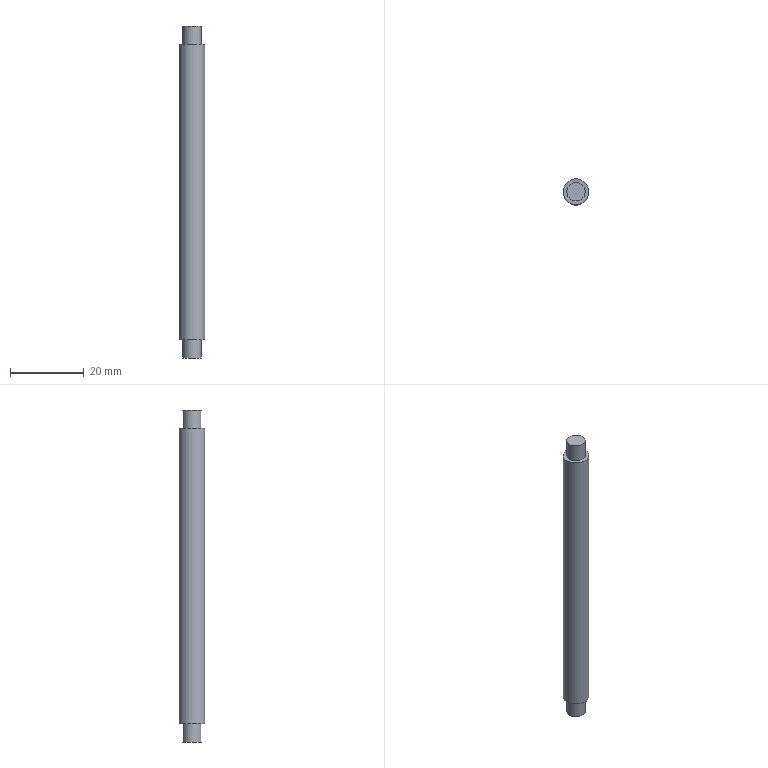Component | NX | STRUT_3 | 1 solid | 7 faces | box 7 x 7 x 90 mm | volume 3275 mm3 | plane 4 | cylinder 3 | commonest cylinder face diameters 5 x2 7 x1
STEP:
#1=CARTESIAN_POINT('',(0.,0.,0.));
#2=DIRECTION('',(0.,0.,1.));
#3=DIRECTION('',(1.,0.,0.));
#4=AXIS2_PLACEMENT_3D('',#1,#2,#3);
#5=CARTESIAN_POINT('',(-7.112,-26.214,-154.808));
#6=VERTEX_POINT('',#5);
#7=CARTESIAN_POINT('',(-9.612,-26.214,-154.808));
#8=DIRECTION('',(0.,0.,1.));
#9=DIRECTION('',(1.,0.,0.));
#10=AXIS2_PLACEMENT_3D('',#7,#8,#9);
#11=CIRCLE('',#10,2.5);
#12=CARTESIAN_POINT('',(-9.612,-26.214,-154.808));
#13=DIRECTION('',(0.,0.,-1.));
#14=DIRECTION('',(-1.,0.,0.));
#15=AXIS2_PLACEMENT_3D('',#12,#13,#14);
#16=PLANE('',#15);
#17=CARTESIAN_POINT('',(-2.5,0.));
#18=CARTESIAN_POINT('',(-2.5,4.33));
#19=CARTESIAN_POINT('',(1.25,2.165));
#20=CARTESIAN_POINT('',(5.,0.));
#21=CARTESIAN_POINT('',(1.25,-2.165));
#22=CARTESIAN_POINT('',(-2.5,-4.33));
#23=CARTESIAN_POINT('',(-2.5,0.));
#24=(BOUNDED_CURVE()B_SPLINE_CURVE(2,(#17,#18,#19,#20,#21,#22,#23),.UNSPECIFIED.,.T.,.F.)B_SPLINE_CURVE_WITH_KNOTS((1,2,2,2,2,1),(-2.094,0.,2.094,4.189,6.283,8.378),.UNSPECIFIED.)CURVE()GEOMETRIC_REPRESENTATION_ITEM()RATIONAL_B_SPLINE_CURVE((1.,0.5,1.,0.5,1.,0.5,1.))REPRESENTATION_ITEM(''));
#25=(GEOMETRIC_REPRESENTATION_CONTEXT(2)PARAMETRIC_REPRESENTATION_CONTEXT()REPRESENTATION_CONTEXT('',''));
#26=DEFINITIONAL_REPRESENTATION('',(#24),#25);
#27=PCURVE('',#16,#26);
#28=CARTESIAN_POINT('',(-9.612,-26.214,-154.808));
#29=DIRECTION('',(0.,0.,1.));
#30=DIRECTION('',(1.,0.,0.));
#31=AXIS2_PLACEMENT_3D('',#28,#29,#30);
#32=CYLINDRICAL_SURFACE('',#31,2.5);
#33=CARTESIAN_POINT('',(0.,0.));
#34=DIRECTION('',(1.,0.));
#35=VECTOR('',#34,1.);
#36=LINE('',#33,#35);
#37=(GEOMETRIC_REPRESENTATION_CONTEXT(2)PARAMETRIC_REPRESENTATION_CONTEXT()REPRESENTATION_CONTEXT('',''));
#38=DEFINITIONAL_REPRESENTATION('',(#36),#37);
#39=PCURVE('',#32,#38);
#40=SURFACE_CURVE('',#11,(#27,#39),.PCURVE_S1.);
#41=EDGE_CURVE('',#6,#6,#40,.T.);
#42=ORIENTED_EDGE('',*,*,#41,.F.);
#43=EDGE_LOOP('',(#42));
#44=FACE_BOUND('',#43,.T.);
#45=ADVANCED_FACE('',(#44),#16,.T.);
#46=CARTESIAN_POINT('',(-7.112,-26.214,-149.808));
#47=VERTEX_POINT('',#46);
#48=CARTESIAN_POINT('',(-12.112,-26.214,-149.808));
#49=VERTEX_POINT('',#48);
#50=CARTESIAN_POINT('',(-9.612,-26.214,-149.808));
#51=DIRECTION('',(0.,0.,1.));
#52=DIRECTION('',(-1.,0.,0.));
#53=AXIS2_PLACEMENT_3D('',#50,#51,#52);
#54=CIRCLE('',#53,2.5);
#55=CARTESIAN_POINT('',(-3.142,5.));
#56=DIRECTION('',(1.,0.));
#57=VECTOR('',#56,1.);
#58=LINE('',#55,#57);
#59=(GEOMETRIC_REPRESENTATION_CONTEXT(2)PARAMETRIC_REPRESENTATION_CONTEXT()REPRESENTATION_CONTEXT('',''));
#60=DEFINITIONAL_REPRESENTATION('',(#58),#59);
#61=PCURVE('',#32,#60);
#62=CARTESIAN_POINT('',(-9.612,-26.214,-149.808));
#63=DIRECTION('',(0.,0.,-1.));
#64=DIRECTION('',(-1.,0.,0.));
#65=AXIS2_PLACEMENT_3D('',#62,#63,#64);
#66=PLANE('',#65);
#67=CARTESIAN_POINT('',(2.5,0.));
#68=CARTESIAN_POINT('',(2.5,-4.33));
#69=CARTESIAN_POINT('',(-1.25,-2.165));
#70=CARTESIAN_POINT('',(-5.,-0.));
#71=CARTESIAN_POINT('',(-1.25,2.165));
#72=CARTESIAN_POINT('',(2.5,4.33));
#73=CARTESIAN_POINT('',(2.5,0.));
#74=(BOUNDED_CURVE()B_SPLINE_CURVE(2,(#67,#68,#69,#70,#71,#72,#73),.UNSPECIFIED.,.T.,.F.)B_SPLINE_CURVE_WITH_KNOTS((1,2,2,2,2,1),(-2.094,0.,2.094,4.189,6.283,8.378),.UNSPECIFIED.)CURVE()GEOMETRIC_REPRESENTATION_ITEM()RATIONAL_B_SPLINE_CURVE((1.,0.5,1.,0.5,1.,0.5,1.))REPRESENTATION_ITEM(''));
#75=(GEOMETRIC_REPRESENTATION_CONTEXT(2)PARAMETRIC_REPRESENTATION_CONTEXT()REPRESENTATION_CONTEXT('',''));
#76=DEFINITIONAL_REPRESENTATION('',(#74),#75);
#77=PCURVE('',#66,#76);
#78=SURFACE_CURVE('',#54,(#61,#77),.PCURVE_S1.);
#79=EDGE_CURVE('',#47,#49,#78,.T.);
#80=ORIENTED_EDGE('',*,*,#79,.F.);
#81=CARTESIAN_POINT('',(-7.112,-26.214,-154.808));
#82=CARTESIAN_POINT('',(-7.112,-26.214,-149.808));
#83=B_SPLINE_CURVE_WITH_KNOTS('',1,(#81,#82),.UNSPECIFIED.,.F.,.F.,(2,2),(0.,5.),.PIECEWISE_BEZIER_KNOTS.);
#84=CARTESIAN_POINT('',(0.,0.));
#85=DIRECTION('',(0.,1.));
#86=VECTOR('',#85,1.);
#87=LINE('',#84,#86);
#88=(GEOMETRIC_REPRESENTATION_CONTEXT(2)PARAMETRIC_REPRESENTATION_CONTEXT()REPRESENTATION_CONTEXT('',''));
#89=DEFINITIONAL_REPRESENTATION('',(#87),#88);
#90=PCURVE('',#32,#89);
#91=CARTESIAN_POINT('',(6.283,0.));
#92=DIRECTION('',(0.,1.));
#93=VECTOR('',#92,1.);
#94=LINE('',#91,#93);
#95=(GEOMETRIC_REPRESENTATION_CONTEXT(2)PARAMETRIC_REPRESENTATION_CONTEXT()REPRESENTATION_CONTEXT('',''));
#96=DEFINITIONAL_REPRESENTATION('',(#94),#95);
#97=PCURVE('',#32,#96);
#98=SEAM_CURVE('',#83,(#90,#97),.PCURVE_S1.);
#99=EDGE_CURVE('',#6,#47,#98,.T.);
#100=ORIENTED_EDGE('',*,*,#99,.F.);
#101=ORIENTED_EDGE('',*,*,#41,.T.);
#102=ORIENTED_EDGE('',*,*,#99,.T.);
#103=CARTESIAN_POINT('',(-9.612,-26.214,-149.808));
#104=DIRECTION('',(0.,0.,1.));
#105=DIRECTION('',(-1.,0.,0.));
#106=AXIS2_PLACEMENT_3D('',#103,#104,#105);
#107=CIRCLE('',#106,2.5);
#108=CARTESIAN_POINT('',(3.142,5.));
#109=DIRECTION('',(1.,0.));
#110=VECTOR('',#109,1.);
#111=LINE('',#108,#110);
#112=(GEOMETRIC_REPRESENTATION_CONTEXT(2)PARAMETRIC_REPRESENTATION_CONTEXT()REPRESENTATION_CONTEXT('',''));
#113=DEFINITIONAL_REPRESENTATION('',(#111),#112);
#114=PCURVE('',#32,#113);
#115=CARTESIAN_POINT('',(2.5,0.));
#116=CARTESIAN_POINT('',(2.5,-4.33));
#117=CARTESIAN_POINT('',(-1.25,-2.165));
#118=CARTESIAN_POINT('',(-5.,-0.));
#119=CARTESIAN_POINT('',(-1.25,2.165));
#120=CARTESIAN_POINT('',(2.5,4.33));
#121=CARTESIAN_POINT('',(2.5,0.));
#122=(BOUNDED_CURVE()B_SPLINE_CURVE(2,(#115,#116,#117,#118,#119,#120,#121),.UNSPECIFIED.,.T.,.F.)B_SPLINE_CURVE_WITH_KNOTS((1,2,2,2,2,1),(-2.094,0.,2.094,4.189,6.283,8.378),.UNSPECIFIED.)CURVE()GEOMETRIC_REPRESENTATION_ITEM()RATIONAL_B_SPLINE_CURVE((1.,0.5,1.,0.5,1.,0.5,1.))REPRESENTATION_ITEM(''));
#123=(GEOMETRIC_REPRESENTATION_CONTEXT(2)PARAMETRIC_REPRESENTATION_CONTEXT()REPRESENTATION_CONTEXT('',''));
#124=DEFINITIONAL_REPRESENTATION('',(#122),#123);
#125=PCURVE('',#66,#124);
#126=SURFACE_CURVE('',#107,(#114,#125),.PCURVE_S1.);
#127=EDGE_CURVE('',#49,#47,#126,.T.);
#128=ORIENTED_EDGE('',*,*,#127,.F.);
#129=EDGE_LOOP('',(#80,#100,#101,#102,#128));
#130=FACE_BOUND('',#129,.T.);
#131=ADVANCED_FACE('',(#130),#32,.T.);
#132=CARTESIAN_POINT('',(-7.112,-26.214,-69.808));
#133=VERTEX_POINT('',#132);
#134=CARTESIAN_POINT('',(-9.612,-26.214,-69.808));
#135=DIRECTION('',(0.,0.,1.));
#136=DIRECTION('',(1.,0.,0.));
#137=AXIS2_PLACEMENT_3D('',#134,#135,#136);
#138=CIRCLE('',#137,2.5);
#139=CARTESIAN_POINT('',(-9.612,-26.214,-69.808));
#140=DIRECTION('',(0.,0.,1.));
#141=DIRECTION('',(1.,0.,0.));
#142=AXIS2_PLACEMENT_3D('',#139,#140,#141);
#143=PLANE('',#142);
#144=CARTESIAN_POINT('',(0.,0.));
#145=DIRECTION('',(1.,0.));
#146=AXIS2_PLACEMENT_2D('',#144,#145);
#147=CIRCLE('',#146,2.5);
#148=(GEOMETRIC_REPRESENTATION_CONTEXT(2)PARAMETRIC_REPRESENTATION_CONTEXT()REPRESENTATION_CONTEXT('',''));
#149=DEFINITIONAL_REPRESENTATION('',(#147),#148);
#150=PCURVE('',#143,#149);
#151=CARTESIAN_POINT('',(-9.612,-26.214,-69.808));
#152=DIRECTION('',(0.,0.,1.));
#153=DIRECTION('',(1.,0.,0.));
#154=AXIS2_PLACEMENT_3D('',#151,#152,#153);
#155=CYLINDRICAL_SURFACE('',#154,2.5);
#156=CARTESIAN_POINT('',(0.,0.));
#157=DIRECTION('',(1.,0.));
#158=VECTOR('',#157,1.);
#159=LINE('',#156,#158);
#160=(GEOMETRIC_REPRESENTATION_CONTEXT(2)PARAMETRIC_REPRESENTATION_CONTEXT()REPRESENTATION_CONTEXT('',''));
#161=DEFINITIONAL_REPRESENTATION('',(#159),#160);
#162=PCURVE('',#155,#161);
#163=SURFACE_CURVE('',#138,(#150,#162),.PCURVE_S1.);
#164=EDGE_CURVE('',#133,#133,#163,.T.);
#165=ORIENTED_EDGE('',*,*,#164,.F.);
#166=EDGE_LOOP('',(#165));
#167=FACE_BOUND('',#166,.T.);
#168=CARTESIAN_POINT('',(-6.112,-26.214,-69.808));
#169=VERTEX_POINT('',#168);
#170=CARTESIAN_POINT('',(-9.612,-26.214,-69.808));
#171=DIRECTION('',(0.,0.,-1.));
#172=DIRECTION('',(1.,0.,0.));
#173=AXIS2_PLACEMENT_3D('',#170,#171,#172);
#174=CIRCLE('',#173,3.5);
#175=CARTESIAN_POINT('',(3.5,0.));
#176=CARTESIAN_POINT('',(3.5,-6.062));
#177=CARTESIAN_POINT('',(-1.75,-3.031));
#178=CARTESIAN_POINT('',(-7.,-0.));
#179=CARTESIAN_POINT('',(-1.75,3.031));
#180=CARTESIAN_POINT('',(3.5,6.062));
#181=CARTESIAN_POINT('',(3.5,0.));
#182=(BOUNDED_CURVE()B_SPLINE_CURVE(2,(#175,#176,#177,#178,#179,#180,#181),.UNSPECIFIED.,.T.,.F.)B_SPLINE_CURVE_WITH_KNOTS((1,2,2,2,2,1),(-2.094,0.,2.094,4.189,6.283,8.378),.UNSPECIFIED.)CURVE()GEOMETRIC_REPRESENTATION_ITEM()RATIONAL_B_SPLINE_CURVE((1.,0.5,1.,0.5,1.,0.5,1.))REPRESENTATION_ITEM(''));
#183=(GEOMETRIC_REPRESENTATION_CONTEXT(2)PARAMETRIC_REPRESENTATION_CONTEXT()REPRESENTATION_CONTEXT('',''));
#184=DEFINITIONAL_REPRESENTATION('',(#182),#183);
#185=PCURVE('',#143,#184);
#186=CARTESIAN_POINT('',(-9.612,-26.214,-149.808));
#187=DIRECTION('',(0.,0.,1.));
#188=DIRECTION('',(1.,0.,0.));
#189=AXIS2_PLACEMENT_3D('',#186,#187,#188);
#190=CYLINDRICAL_SURFACE('',#189,3.5);
#191=CARTESIAN_POINT('',(6.283,80.));
#192=DIRECTION('',(-1.,0.));
#193=VECTOR('',#192,1.);
#194=LINE('',#191,#193);
#195=(GEOMETRIC_REPRESENTATION_CONTEXT(2)PARAMETRIC_REPRESENTATION_CONTEXT()REPRESENTATION_CONTEXT('',''));
#196=DEFINITIONAL_REPRESENTATION('',(#194),#195);
#197=PCURVE('',#190,#196);
#198=SURFACE_CURVE('',#174,(#185,#197),.PCURVE_S1.);
#199=EDGE_CURVE('',#169,#169,#198,.T.);
#200=ORIENTED_EDGE('',*,*,#199,.F.);
#201=EDGE_LOOP('',(#200));
#202=FACE_BOUND('',#201,.T.);
#203=ADVANCED_FACE('',(#167,#202),#143,.T.);
#204=ORIENTED_EDGE('',*,*,#127,.T.);
#205=ORIENTED_EDGE('',*,*,#79,.T.);
#206=EDGE_LOOP('',(#204,#205));
#207=FACE_BOUND('',#206,.T.);
#208=CARTESIAN_POINT('',(-6.112,-26.214,-149.808));
#209=VERTEX_POINT('',#208);
#210=CARTESIAN_POINT('',(-9.612,-26.214,-149.808));
#211=DIRECTION('',(0.,0.,1.));
#212=DIRECTION('',(1.,0.,0.));
#213=AXIS2_PLACEMENT_3D('',#210,#211,#212);
#214=CIRCLE('',#213,3.5);
#215=CARTESIAN_POINT('',(-3.5,0.));
#216=CARTESIAN_POINT('',(-3.5,6.062));
#217=CARTESIAN_POINT('',(1.75,3.031));
#218=CARTESIAN_POINT('',(7.,0.));
#219=CARTESIAN_POINT('',(1.75,-3.031));
#220=CARTESIAN_POINT('',(-3.5,-6.062));
#221=CARTESIAN_POINT('',(-3.5,0.));
#222=(BOUNDED_CURVE()B_SPLINE_CURVE(2,(#215,#216,#217,#218,#219,#220,#221),.UNSPECIFIED.,.T.,.F.)B_SPLINE_CURVE_WITH_KNOTS((1,2,2,2,2,1),(-2.094,0.,2.094,4.189,6.283,8.378),.UNSPECIFIED.)CURVE()GEOMETRIC_REPRESENTATION_ITEM()RATIONAL_B_SPLINE_CURVE((1.,0.5,1.,0.5,1.,0.5,1.))REPRESENTATION_ITEM(''));
#223=(GEOMETRIC_REPRESENTATION_CONTEXT(2)PARAMETRIC_REPRESENTATION_CONTEXT()REPRESENTATION_CONTEXT('',''));
#224=DEFINITIONAL_REPRESENTATION('',(#222),#223);
#225=PCURVE('',#66,#224);
#226=CARTESIAN_POINT('',(0.,0.));
#227=DIRECTION('',(1.,0.));
#228=VECTOR('',#227,1.);
#229=LINE('',#226,#228);
#230=(GEOMETRIC_REPRESENTATION_CONTEXT(2)PARAMETRIC_REPRESENTATION_CONTEXT()REPRESENTATION_CONTEXT('',''));
#231=DEFINITIONAL_REPRESENTATION('',(#229),#230);
#232=PCURVE('',#190,#231);
#233=SURFACE_CURVE('',#214,(#225,#232),.PCURVE_S1.);
#234=EDGE_CURVE('',#209,#209,#233,.T.);
#235=ORIENTED_EDGE('',*,*,#234,.F.);
#236=EDGE_LOOP('',(#235));
#237=FACE_BOUND('',#236,.T.);
#238=ADVANCED_FACE('',(#207,#237),#66,.T.);
#239=ORIENTED_EDGE('',*,*,#199,.T.);
#240=CARTESIAN_POINT('',(-6.112,-26.214,-149.808));
#241=CARTESIAN_POINT('',(-6.112,-26.214,-69.808));
#242=B_SPLINE_CURVE_WITH_KNOTS('',1,(#240,#241),.UNSPECIFIED.,.F.,.F.,(2,2),(0.,80.),.PIECEWISE_BEZIER_KNOTS.);
#243=CARTESIAN_POINT('',(0.,0.));
#244=DIRECTION('',(0.,1.));
#245=VECTOR('',#244,1.);
#246=LINE('',#243,#245);
#247=(GEOMETRIC_REPRESENTATION_CONTEXT(2)PARAMETRIC_REPRESENTATION_CONTEXT()REPRESENTATION_CONTEXT('',''));
#248=DEFINITIONAL_REPRESENTATION('',(#246),#247);
#249=PCURVE('',#190,#248);
#250=CARTESIAN_POINT('',(6.283,0.));
#251=DIRECTION('',(0.,1.));
#252=VECTOR('',#251,1.);
#253=LINE('',#250,#252);
#254=(GEOMETRIC_REPRESENTATION_CONTEXT(2)PARAMETRIC_REPRESENTATION_CONTEXT()REPRESENTATION_CONTEXT('',''));
#255=DEFINITIONAL_REPRESENTATION('',(#253),#254);
#256=PCURVE('',#190,#255);
#257=SEAM_CURVE('',#242,(#249,#256),.PCURVE_S1.);
#258=EDGE_CURVE('',#209,#169,#257,.T.);
#259=ORIENTED_EDGE('',*,*,#258,.F.);
#260=ORIENTED_EDGE('',*,*,#234,.T.);
#261=ORIENTED_EDGE('',*,*,#258,.T.);
#262=EDGE_LOOP('',(#239,#259,#260,#261));
#263=FACE_BOUND('',#262,.T.);
#264=ADVANCED_FACE('',(#263),#190,.T.);
#265=CARTESIAN_POINT('',(-7.112,-26.214,-64.808));
#266=VERTEX_POINT('',#265);
#267=CARTESIAN_POINT('',(-9.612,-26.214,-64.808));
#268=DIRECTION('',(0.,0.,-1.));
#269=DIRECTION('',(1.,0.,0.));
#270=AXIS2_PLACEMENT_3D('',#267,#268,#269);
#271=CIRCLE('',#270,2.5);
#272=CARTESIAN_POINT('',(-9.612,-26.214,-64.808));
#273=DIRECTION('',(0.,0.,1.));
#274=DIRECTION('',(1.,0.,0.));
#275=AXIS2_PLACEMENT_3D('',#272,#273,#274);
#276=PLANE('',#275);
#277=CARTESIAN_POINT('',(2.5,0.));
#278=CARTESIAN_POINT('',(2.5,-4.33));
#279=CARTESIAN_POINT('',(-1.25,-2.165));
#280=CARTESIAN_POINT('',(-5.,-0.));
#281=CARTESIAN_POINT('',(-1.25,2.165));
#282=CARTESIAN_POINT('',(2.5,4.33));
#283=CARTESIAN_POINT('',(2.5,0.));
#284=(BOUNDED_CURVE()B_SPLINE_CURVE(2,(#277,#278,#279,#280,#281,#282,#283),.UNSPECIFIED.,.T.,.F.)B_SPLINE_CURVE_WITH_KNOTS((1,2,2,2,2,1),(-2.094,0.,2.094,4.189,6.283,8.378),.UNSPECIFIED.)CURVE()GEOMETRIC_REPRESENTATION_ITEM()RATIONAL_B_SPLINE_CURVE((1.,0.5,1.,0.5,1.,0.5,1.))REPRESENTATION_ITEM(''));
#285=(GEOMETRIC_REPRESENTATION_CONTEXT(2)PARAMETRIC_REPRESENTATION_CONTEXT()REPRESENTATION_CONTEXT('',''));
#286=DEFINITIONAL_REPRESENTATION('',(#284),#285);
#287=PCURVE('',#276,#286);
#288=CARTESIAN_POINT('',(6.283,5.));
#289=DIRECTION('',(-1.,0.));
#290=VECTOR('',#289,1.);
#291=LINE('',#288,#290);
#292=(GEOMETRIC_REPRESENTATION_CONTEXT(2)PARAMETRIC_REPRESENTATION_CONTEXT()REPRESENTATION_CONTEXT('',''));
#293=DEFINITIONAL_REPRESENTATION('',(#291),#292);
#294=PCURVE('',#155,#293);
#295=SURFACE_CURVE('',#271,(#287,#294),.PCURVE_S1.);
#296=EDGE_CURVE('',#266,#266,#295,.T.);
#297=ORIENTED_EDGE('',*,*,#296,.F.);
#298=EDGE_LOOP('',(#297));
#299=FACE_BOUND('',#298,.T.);
#300=ADVANCED_FACE('',(#299),#276,.T.);
#301=ORIENTED_EDGE('',*,*,#296,.T.);
#302=CARTESIAN_POINT('',(-7.112,-26.214,-69.808));
#303=CARTESIAN_POINT('',(-7.112,-26.214,-64.808));
#304=B_SPLINE_CURVE_WITH_KNOTS('',1,(#302,#303),.UNSPECIFIED.,.F.,.F.,(2,2),(0.,5.),.PIECEWISE_BEZIER_KNOTS.);
#305=CARTESIAN_POINT('',(0.,0.));
#306=DIRECTION('',(0.,1.));
#307=VECTOR('',#306,1.);
#308=LINE('',#305,#307);
#309=(GEOMETRIC_REPRESENTATION_CONTEXT(2)PARAMETRIC_REPRESENTATION_CONTEXT()REPRESENTATION_CONTEXT('',''));
#310=DEFINITIONAL_REPRESENTATION('',(#308),#309);
#311=PCURVE('',#155,#310);
#312=CARTESIAN_POINT('',(6.283,0.));
#313=DIRECTION('',(0.,1.));
#314=VECTOR('',#313,1.);
#315=LINE('',#312,#314);
#316=(GEOMETRIC_REPRESENTATION_CONTEXT(2)PARAMETRIC_REPRESENTATION_CONTEXT()REPRESENTATION_CONTEXT('',''));
#317=DEFINITIONAL_REPRESENTATION('',(#315),#316);
#318=PCURVE('',#155,#317);
#319=SEAM_CURVE('',#304,(#311,#318),.PCURVE_S1.);
#320=EDGE_CURVE('',#133,#266,#319,.T.);
#321=ORIENTED_EDGE('',*,*,#320,.F.);
#322=ORIENTED_EDGE('',*,*,#164,.T.);
#323=ORIENTED_EDGE('',*,*,#320,.T.);
#324=EDGE_LOOP('',(#301,#321,#322,#323));
#325=FACE_BOUND('',#324,.T.);
#326=ADVANCED_FACE('',(#325),#155,.T.);
#327=CLOSED_SHELL('',(#45,#131,#203,#238,#264,#300,#326));
#328=MANIFOLD_SOLID_BREP('',#327);
#329=(LENGTH_UNIT()NAMED_UNIT(*)SI_UNIT(.MILLI.,.METRE.));
#330=UNCERTAINTY_MEASURE_WITH_UNIT(LENGTH_MEASURE(0.000005),#329,'','');
#331=(NAMED_UNIT(*)PLANE_ANGLE_UNIT()SI_UNIT($,.RADIAN.));
#332=(NAMED_UNIT(*)SI_UNIT($,.STERADIAN.)SOLID_ANGLE_UNIT());
#333=(GEOMETRIC_REPRESENTATION_CONTEXT(3)GLOBAL_UNCERTAINTY_ASSIGNED_CONTEXT((#330))GLOBAL_UNIT_ASSIGNED_CONTEXT((#329,#331,#332))REPRESENTATION_CONTEXT('',''));
#334=ADVANCED_BREP_SHAPE_REPRESENTATION('',(#4,#328),#333);